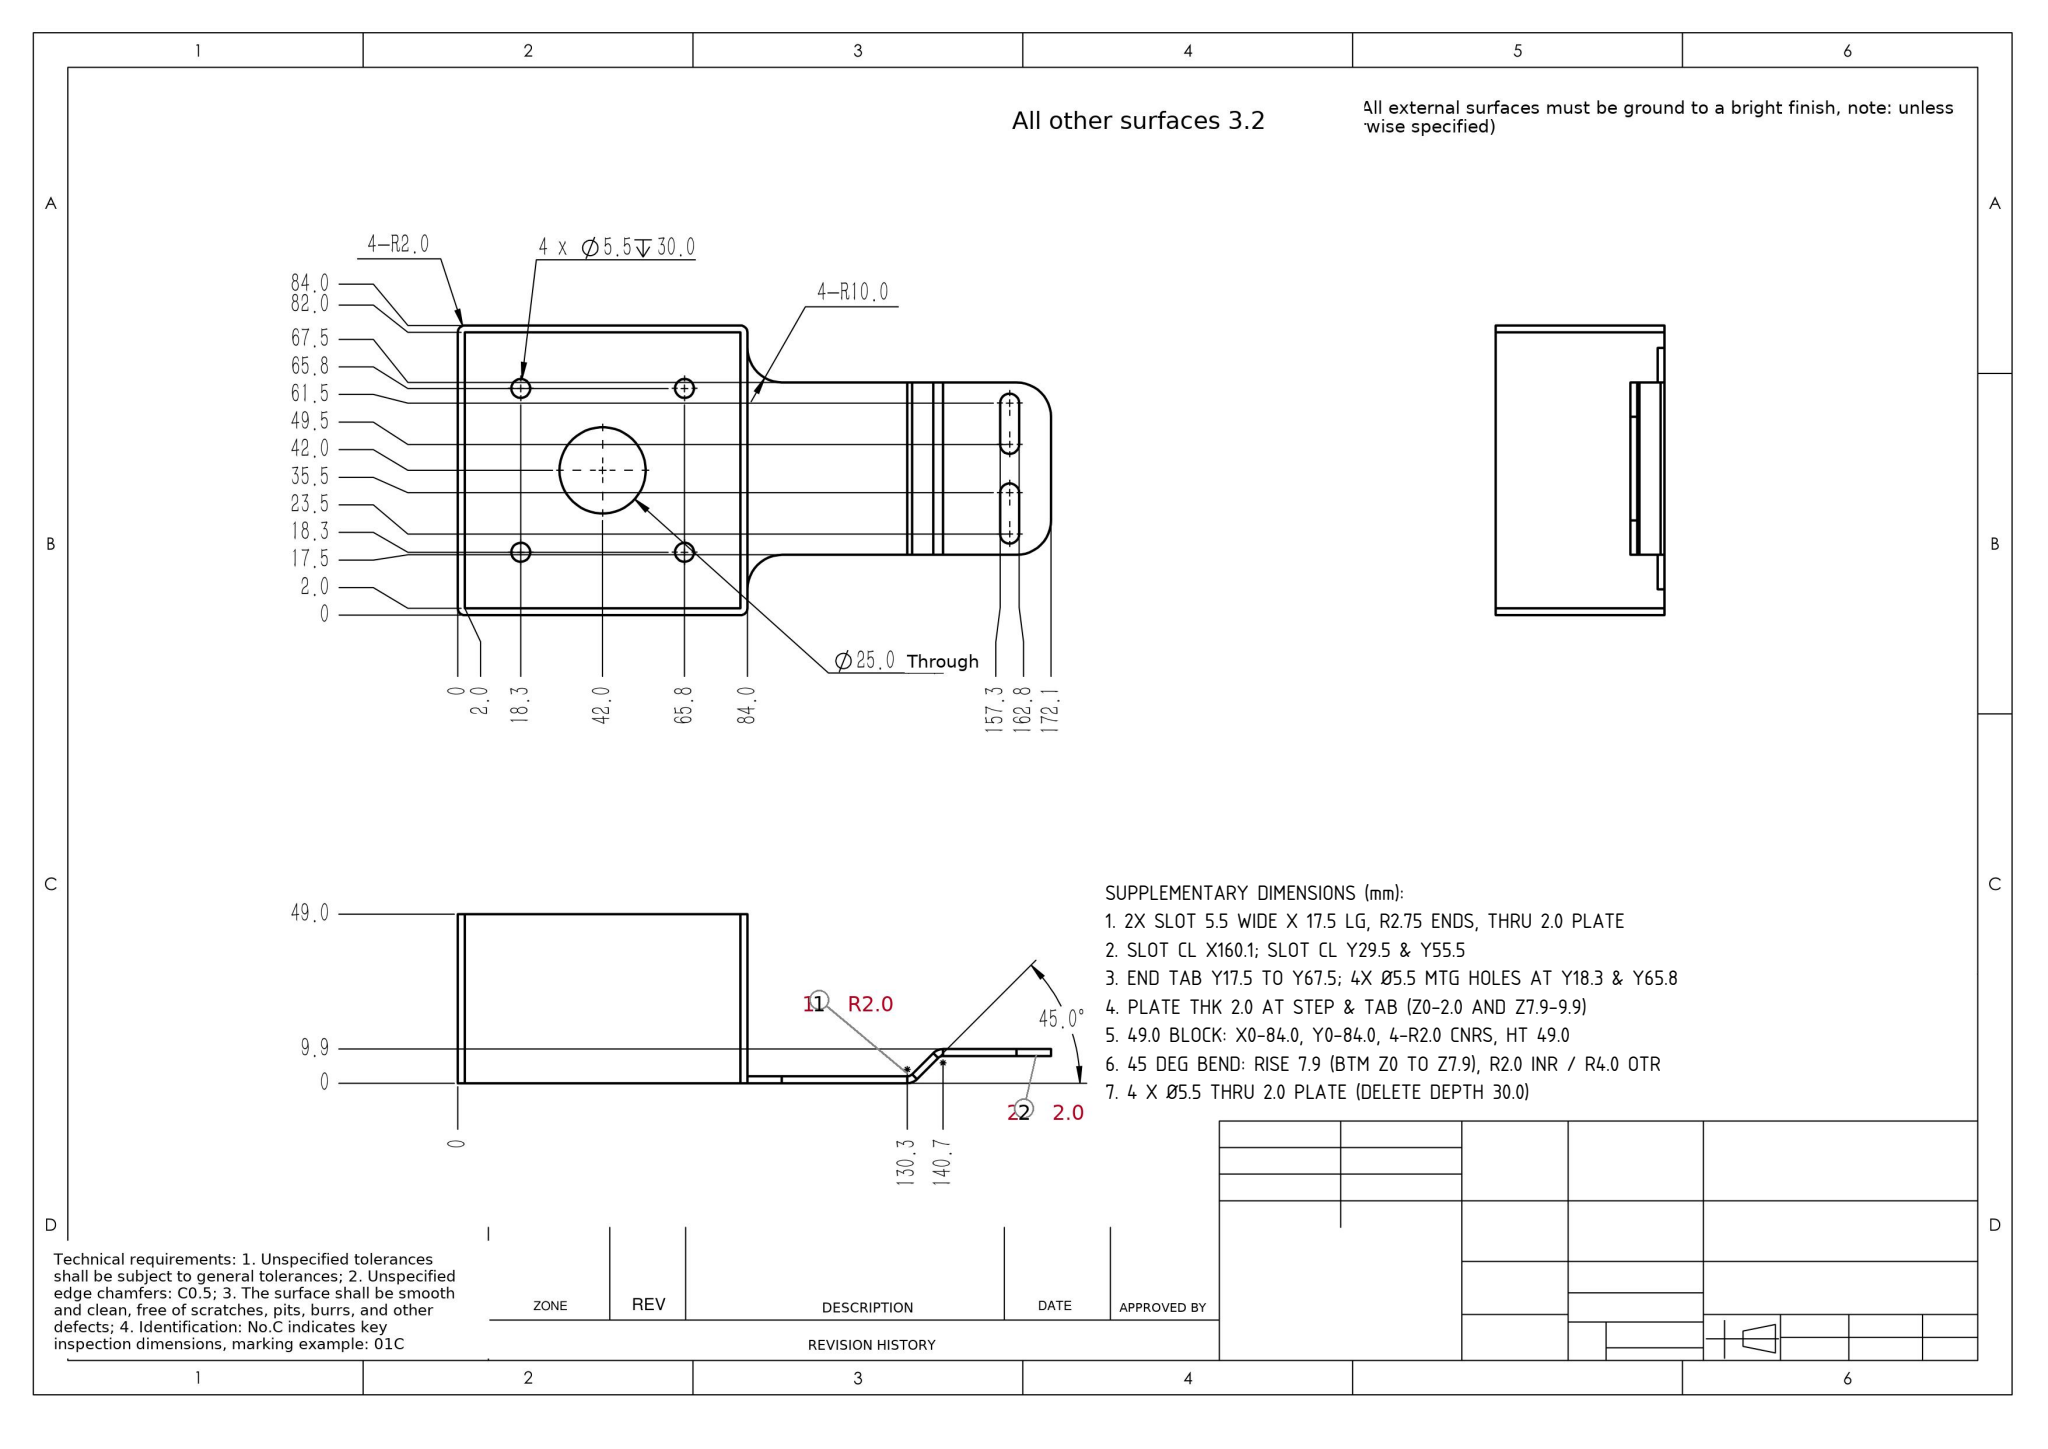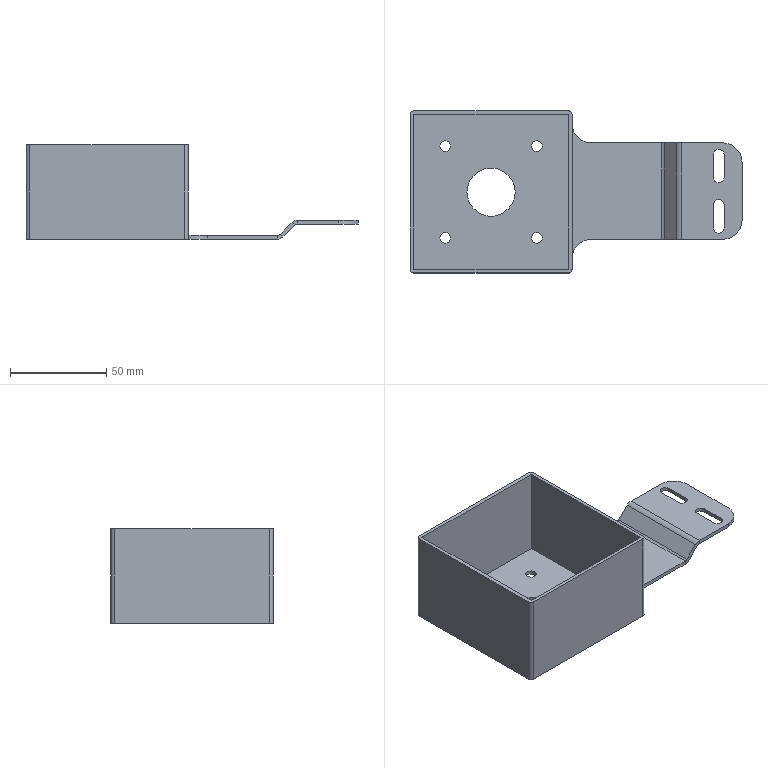Part | SolidWorks | mm | 1 solid | 57 faces | box 172.07 x 84 x 49 mm | volume 52353 mm3 | plane 31 | cylinder 26 | commonest cylinder face diameters 5.5 x12 4 x6 20 x4 25 x2 8 x2